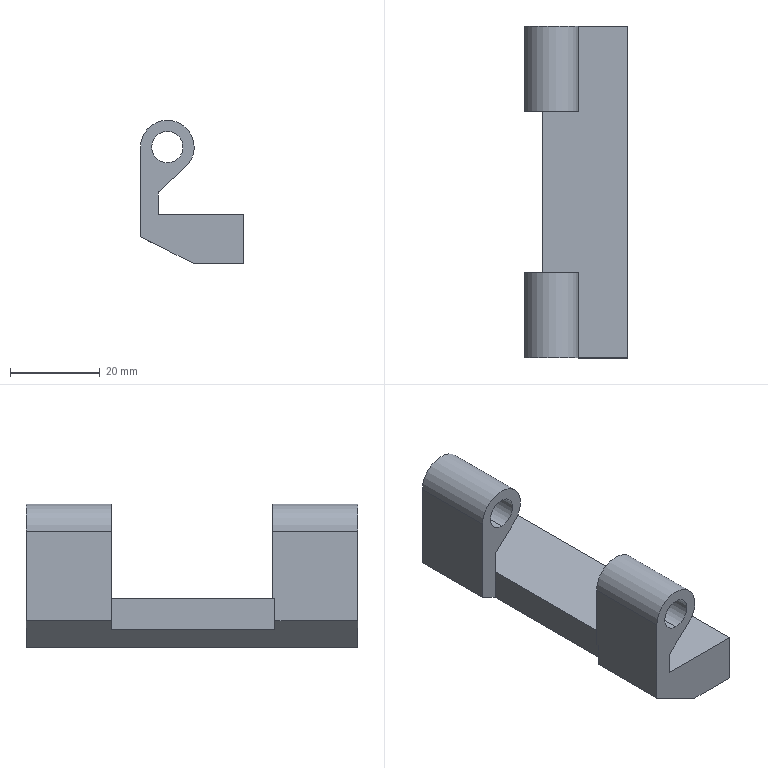Component | SolidWorks | 201LargeHinge-5 | 1 solid | 55 faces | volume 14291 mm3 | plane 34 | cylinder 21 | commonest cylinder face diameters 10 x9 6 x6 7 x4 12 x2